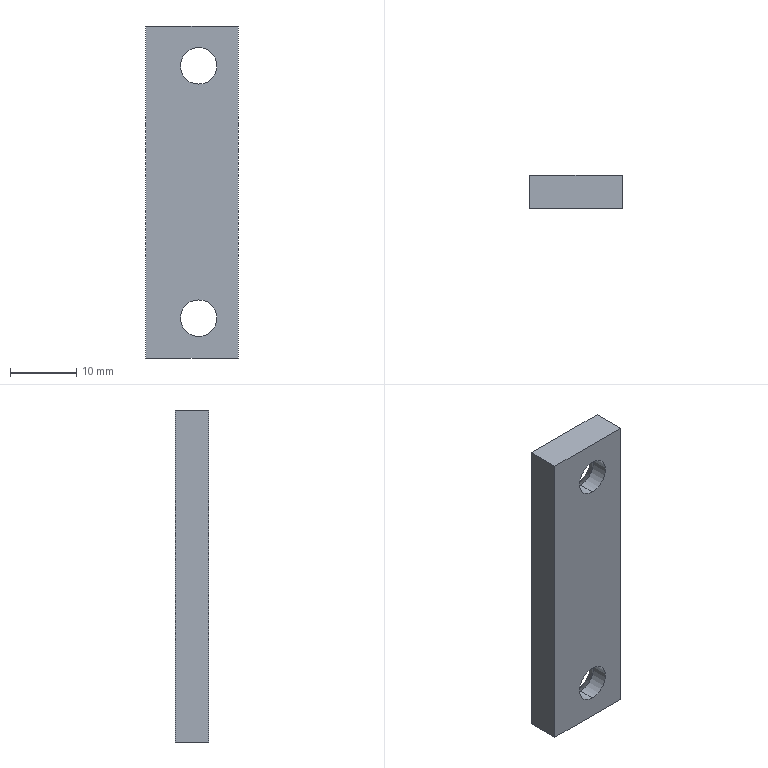Component | SolidWorks | PusherBlockSlideSeatCoverPlate3-1 | 1 solid | 14 faces | box 14 x 5 x 50 mm | volume 3128 mm3 | plane 6 | cone 4 | cylinder 4 | commonest cylinder face diameters 5.5 x4
build123d program:
from build123d import *

# Parameters (mm, degrees)
SKETCH1_W                                    = 50
SKETCH1_H                                    = 14
BOSS_EXTRUDE1_DEPTH                          = 5
TAPERED_COUNTERSUNK_HOLE_FOR_M5_FLAT_2_COUNT = 2
TAPERED_COUNTERSUNK_HOLE_FOR_M5_FLAT_2_PITCH = 38


with BuildPart() as part:
    # Sketch1 → Boss-Extrude1 (new body)
    with BuildSketch(Plane.XY):
        with Locations((-25, 7)):
            Rectangle(SKETCH1_W, SKETCH1_H)
    extrude(amount=BOSS_EXTRUDE1_DEPTH)

    # Sketch2 → Tapered Countersunk Hole for M5 Flat Hea (revolve, cut)
    with BuildSketch(Plane(origin=(-44, 6, 5), x_dir=(0, -1, 0), z_dir=(1, 0, 0))):
        Polygon((0, 0), (0, 5), (2.75, 5), (2.75, 2.45), (5.2, 0), align=None)
    tapered_countersunk_hole_for_m5_flat_hea = revolve(axis=Axis((-44, 6, 11.35), (0, 0, -1)), mode=Mode.SUBTRACT)

    # Tapered Countersunk Hole for M5 Flat 2: Tapered Countersunk Hole for M5 Flat Hea ×2
    with Locations(*[(i * TAPERED_COUNTERSUNK_HOLE_FOR_M5_FLAT_2_PITCH, 0, 0) for i in range(1, TAPERED_COUNTERSUNK_HOLE_FOR_M5_FLAT_2_COUNT)]):
        add(tapered_countersunk_hole_for_m5_flat_hea, mode=Mode.SUBTRACT)


solid = part.part

# Placed as in the assembly
solid = solid.moved(Location((22.085, 11.195, 51.579), (-90, 0, 90)))
STEP:
#1=COLOUR_RGB('',0.7922,0.8196,0.9333);
#2=FILL_AREA_STYLE_COLOUR('',#1);
#3=FILL_AREA_STYLE('',(#2));
#4=SURFACE_STYLE_FILL_AREA(#3);
#5=SURFACE_SIDE_STYLE('',(#4));
#6=SURFACE_STYLE_USAGE(.BOTH.,#5);
#7=PRESENTATION_STYLE_ASSIGNMENT((#6));
#8=CARTESIAN_POINT('',(0.6333,0.5411,3.871));
#9=VERTEX_POINT('',#8);
#10=CARTESIAN_POINT('',(0.6333,0.5411,3.655));
#11=VERTEX_POINT('',#10);
#12=CARTESIAN_POINT('',(0.6333,0.5411,3.763));
#13=DIRECTION('',(-0.,1.,-0.));
#14=DIRECTION('',(0.,0.,-1.));
#15=AXIS2_PLACEMENT_3D('',#12,#13,#14);
#16=CIRCLE('',#15,0.1083);
#17=EDGE_CURVE('',#9,#11,#16,.T.);
#18=ORIENTED_EDGE('',*,*,#17,.F.);
#19=CARTESIAN_POINT('',(0.6333,0.6376,3.968));
#20=VERTEX_POINT('',#19);
#21=CARTESIAN_POINT('',(0.6333,0.6376,3.968));
#22=DIRECTION('',(-0.,0.7071,0.7071));
#23=VECTOR('',#22,39.37);
#24=LINE('',#21,#23);
#25=EDGE_CURVE('',#9,#20,#24,.T.);
#26=ORIENTED_EDGE('',*,*,#25,.T.);
#27=CARTESIAN_POINT('',(0.6333,0.6376,3.558));
#28=VERTEX_POINT('',#27);
#29=CARTESIAN_POINT('',(0.6333,0.6376,3.763));
#30=DIRECTION('',(-0.,1.,-0.));
#31=DIRECTION('',(0.,0.,-1.));
#32=AXIS2_PLACEMENT_3D('',#29,#30,#31);
#33=CIRCLE('',#32,0.2047);
#34=EDGE_CURVE('',#20,#28,#33,.T.);
#35=ORIENTED_EDGE('',*,*,#34,.T.);
#36=CARTESIAN_POINT('',(0.6333,0.6376,3.558));
#37=DIRECTION('',(-0.,0.7071,-0.7071));
#38=VECTOR('',#37,39.37);
#39=LINE('',#36,#38);
#40=EDGE_CURVE('',#11,#28,#39,.T.);
#41=ORIENTED_EDGE('',*,*,#40,.F.);
#42=EDGE_LOOP('',(#18,#26,#35,#41));
#43=FACE_OUTER_BOUND('',#42,.T.);
#44=CARTESIAN_POINT('',(0.6333,0.6376,3.763));
#45=DIRECTION('',(-0.,1.,-0.));
#46=DIRECTION('',(0.,0.,-1.));
#47=AXIS2_PLACEMENT_3D('',#44,#45,#46);
#48=CONICAL_SURFACE('',#47,0.2047,0.7854);
#49=ADVANCED_FACE('',(#43),#48,.F.);
#50=CARTESIAN_POINT('',(0.6333,0.4407,3.871));
#51=VERTEX_POINT('',#50);
#52=CARTESIAN_POINT('',(0.6333,0.4407,3.655));
#53=VERTEX_POINT('',#52);
#54=CARTESIAN_POINT('',(0.6333,0.4407,3.763));
#55=DIRECTION('',(-0.,1.,-0.));
#56=DIRECTION('',(0.,0.,-1.));
#57=AXIS2_PLACEMENT_3D('',#54,#55,#56);
#58=CIRCLE('',#57,0.1083);
#59=EDGE_CURVE('',#51,#53,#58,.T.);
#60=ORIENTED_EDGE('',*,*,#59,.F.);
#61=CARTESIAN_POINT('',(0.6333,0.6376,3.871));
#62=DIRECTION('',(-0.,1.,-0.));
#63=VECTOR('',#62,39.37);
#64=LINE('',#61,#63);
#65=EDGE_CURVE('',#51,#9,#64,.T.);
#66=ORIENTED_EDGE('',*,*,#65,.T.);
#67=ORIENTED_EDGE('',*,*,#17,.T.);
#68=CARTESIAN_POINT('',(0.6333,0.6376,3.655));
#69=DIRECTION('',(-0.,1.,-0.));
#70=VECTOR('',#69,39.37);
#71=LINE('',#68,#70);
#72=EDGE_CURVE('',#53,#11,#71,.T.);
#73=ORIENTED_EDGE('',*,*,#72,.F.);
#74=EDGE_LOOP('',(#60,#66,#67,#73));
#75=FACE_OUTER_BOUND('',#74,.T.);
#76=CARTESIAN_POINT('',(0.6333,0.6376,3.763));
#77=DIRECTION('',(-0.,1.,-0.));
#78=DIRECTION('',(0.,0.,-1.));
#79=AXIS2_PLACEMENT_3D('',#76,#77,#78);
#80=CYLINDRICAL_SURFACE('',#79,0.1083);
#81=ADVANCED_FACE('',(#75),#80,.F.);
#82=CARTESIAN_POINT('',(0.6333,0.5411,2.375));
#83=VERTEX_POINT('',#82);
#84=CARTESIAN_POINT('',(0.6333,0.5411,2.159));
#85=VERTEX_POINT('',#84);
#86=CARTESIAN_POINT('',(0.6333,0.5411,2.267));
#87=DIRECTION('',(-0.,1.,-0.));
#88=DIRECTION('',(0.,0.,-1.));
#89=AXIS2_PLACEMENT_3D('',#86,#87,#88);
#90=CIRCLE('',#89,0.1083);
#91=EDGE_CURVE('',#83,#85,#90,.T.);
#92=ORIENTED_EDGE('',*,*,#91,.F.);
#93=CARTESIAN_POINT('',(0.6333,0.6376,2.472));
#94=VERTEX_POINT('',#93);
#95=CARTESIAN_POINT('',(0.6333,0.6376,2.472));
#96=DIRECTION('',(-0.,0.7071,0.7071));
#97=VECTOR('',#96,39.37);
#98=LINE('',#95,#97);
#99=EDGE_CURVE('',#83,#94,#98,.T.);
#100=ORIENTED_EDGE('',*,*,#99,.T.);
#101=CARTESIAN_POINT('',(0.6333,0.6376,2.062));
#102=VERTEX_POINT('',#101);
#103=CARTESIAN_POINT('',(0.6333,0.6376,2.267));
#104=DIRECTION('',(-0.,1.,-0.));
#105=DIRECTION('',(0.,0.,-1.));
#106=AXIS2_PLACEMENT_3D('',#103,#104,#105);
#107=CIRCLE('',#106,0.2047);
#108=EDGE_CURVE('',#94,#102,#107,.T.);
#109=ORIENTED_EDGE('',*,*,#108,.T.);
#110=CARTESIAN_POINT('',(0.6333,0.6376,2.062));
#111=DIRECTION('',(-0.,0.7071,-0.7071));
#112=VECTOR('',#111,39.37);
#113=LINE('',#110,#112);
#114=EDGE_CURVE('',#85,#102,#113,.T.);
#115=ORIENTED_EDGE('',*,*,#114,.F.);
#116=EDGE_LOOP('',(#92,#100,#109,#115));
#117=FACE_OUTER_BOUND('',#116,.T.);
#118=CARTESIAN_POINT('',(0.6333,0.6376,2.267));
#119=DIRECTION('',(-0.,1.,-0.));
#120=DIRECTION('',(0.,0.,-1.));
#121=AXIS2_PLACEMENT_3D('',#118,#119,#120);
#122=CONICAL_SURFACE('',#121,0.2047,0.7854);
#123=ADVANCED_FACE('',(#117),#122,.F.);
#124=CARTESIAN_POINT('',(0.6333,0.4407,2.375));
#125=VERTEX_POINT('',#124);
#126=CARTESIAN_POINT('',(0.6333,0.4407,2.159));
#127=VERTEX_POINT('',#126);
#128=CARTESIAN_POINT('',(0.6333,0.4407,2.267));
#129=DIRECTION('',(-0.,1.,-0.));
#130=DIRECTION('',(0.,0.,-1.));
#131=AXIS2_PLACEMENT_3D('',#128,#129,#130);
#132=CIRCLE('',#131,0.1083);
#133=EDGE_CURVE('',#125,#127,#132,.T.);
#134=ORIENTED_EDGE('',*,*,#133,.F.);
#135=CARTESIAN_POINT('',(0.6333,0.6376,2.375));
#136=DIRECTION('',(-0.,1.,-0.));
#137=VECTOR('',#136,39.37);
#138=LINE('',#135,#137);
#139=EDGE_CURVE('',#125,#83,#138,.T.);
#140=ORIENTED_EDGE('',*,*,#139,.T.);
#141=ORIENTED_EDGE('',*,*,#91,.T.);
#142=CARTESIAN_POINT('',(0.6333,0.6376,2.159));
#143=DIRECTION('',(-0.,1.,-0.));
#144=VECTOR('',#143,39.37);
#145=LINE('',#142,#144);
#146=EDGE_CURVE('',#127,#85,#145,.T.);
#147=ORIENTED_EDGE('',*,*,#146,.F.);
#148=EDGE_LOOP('',(#134,#140,#141,#147));
#149=FACE_OUTER_BOUND('',#148,.T.);
#150=CARTESIAN_POINT('',(0.6333,0.6376,2.267));
#151=DIRECTION('',(-0.,1.,-0.));
#152=DIRECTION('',(0.,0.,-1.));
#153=AXIS2_PLACEMENT_3D('',#150,#151,#152);
#154=CYLINDRICAL_SURFACE('',#153,0.1083);
#155=ADVANCED_FACE('',(#149),#154,.F.);
#156=CARTESIAN_POINT('',(0.8695,0.4407,2.031));
#157=VERTEX_POINT('',#156);
#158=CARTESIAN_POINT('',(0.3183,0.4407,2.031));
#159=VERTEX_POINT('',#158);
#160=CARTESIAN_POINT('',(0.8695,0.4407,2.031));
#161=DIRECTION('',(-1.,0.,0.));
#162=VECTOR('',#161,39.37);
#163=LINE('',#160,#162);
#164=EDGE_CURVE('',#157,#159,#163,.T.);
#165=ORIENTED_EDGE('',*,*,#164,.T.);
#166=CARTESIAN_POINT('',(0.3183,0.6376,2.031));
#167=VERTEX_POINT('',#166);
#168=CARTESIAN_POINT('',(0.3183,0.6376,2.031));
#169=DIRECTION('',(0.,-1.,0.));
#170=VECTOR('',#169,39.37);
#171=LINE('',#168,#170);
#172=EDGE_CURVE('',#167,#159,#171,.T.);
#173=ORIENTED_EDGE('',*,*,#172,.F.);
#174=CARTESIAN_POINT('',(0.8695,0.6376,2.031));
#175=VERTEX_POINT('',#174);
#176=CARTESIAN_POINT('',(0.8695,0.6376,2.031));
#177=DIRECTION('',(-1.,0.,0.));
#178=VECTOR('',#177,39.37);
#179=LINE('',#176,#178);
#180=EDGE_CURVE('',#175,#167,#179,.T.);
#181=ORIENTED_EDGE('',*,*,#180,.F.);
#182=CARTESIAN_POINT('',(0.8695,0.6376,2.031));
#183=DIRECTION('',(0.,-1.,0.));
#184=VECTOR('',#183,39.37);
#185=LINE('',#182,#184);
#186=EDGE_CURVE('',#175,#157,#185,.T.);
#187=ORIENTED_EDGE('',*,*,#186,.T.);
#188=EDGE_LOOP('',(#165,#173,#181,#187));
#189=FACE_OUTER_BOUND('',#188,.T.);
#190=CARTESIAN_POINT('',(0.8695,0.6376,2.031));
#191=DIRECTION('',(0.,0.,1.));
#192=DIRECTION('',(-0.,1.,-0.));
#193=AXIS2_PLACEMENT_3D('',#190,#191,#192);
#194=PLANE('',#193);
#195=ADVANCED_FACE('',(#189),#194,.F.);
#196=CARTESIAN_POINT('',(0.3183,0.4407,3.999));
#197=VERTEX_POINT('',#196);
#198=CARTESIAN_POINT('',(0.3183,0.4407,2.031));
#199=DIRECTION('',(0.,-0.,1.));
#200=VECTOR('',#199,39.37);
#201=LINE('',#198,#200);
#202=EDGE_CURVE('',#159,#197,#201,.T.);
#203=ORIENTED_EDGE('',*,*,#202,.T.);
#204=CARTESIAN_POINT('',(0.3183,0.6376,3.999));
#205=VERTEX_POINT('',#204);
#206=CARTESIAN_POINT('',(0.3183,0.6376,3.999));
#207=DIRECTION('',(0.,-1.,0.));
#208=VECTOR('',#207,39.37);
#209=LINE('',#206,#208);
#210=EDGE_CURVE('',#205,#197,#209,.T.);
#211=ORIENTED_EDGE('',*,*,#210,.F.);
#212=CARTESIAN_POINT('',(0.3183,0.6376,2.031));
#213=DIRECTION('',(0.,-0.,1.));
#214=VECTOR('',#213,39.37);
#215=LINE('',#212,#214);
#216=EDGE_CURVE('',#167,#205,#215,.T.);
#217=ORIENTED_EDGE('',*,*,#216,.F.);
#218=ORIENTED_EDGE('',*,*,#172,.T.);
#219=EDGE_LOOP('',(#203,#211,#217,#218));
#220=FACE_OUTER_BOUND('',#219,.T.);
#221=CARTESIAN_POINT('',(0.3183,0.6376,2.031));
#222=DIRECTION('',(1.,-0.,-0.));
#223=DIRECTION('',(-0.,0.,-1.));
#224=AXIS2_PLACEMENT_3D('',#221,#222,#223);
#225=PLANE('',#224);
#226=ADVANCED_FACE('',(#220),#225,.F.);
#227=CARTESIAN_POINT('',(0.8695,0.4407,3.999));
#228=VERTEX_POINT('',#227);
#229=CARTESIAN_POINT('',(0.8695,0.4407,3.999));
#230=DIRECTION('',(1.,-0.,-0.));
#231=VECTOR('',#230,39.37);
#232=LINE('',#229,#231);
#233=EDGE_CURVE('',#197,#228,#232,.T.);
#234=ORIENTED_EDGE('',*,*,#233,.T.);
#235=CARTESIAN_POINT('',(0.8695,0.6376,3.999));
#236=VERTEX_POINT('',#235);
#237=CARTESIAN_POINT('',(0.8695,0.6376,3.999));
#238=DIRECTION('',(0.,-1.,0.));
#239=VECTOR('',#238,39.37);
#240=LINE('',#237,#239);
#241=EDGE_CURVE('',#236,#228,#240,.T.);
#242=ORIENTED_EDGE('',*,*,#241,.F.);
#243=CARTESIAN_POINT('',(0.8695,0.6376,3.999));
#244=DIRECTION('',(1.,-0.,-0.));
#245=VECTOR('',#244,39.37);
#246=LINE('',#243,#245);
#247=EDGE_CURVE('',#205,#236,#246,.T.);
#248=ORIENTED_EDGE('',*,*,#247,.F.);
#249=ORIENTED_EDGE('',*,*,#210,.T.);
#250=EDGE_LOOP('',(#234,#242,#248,#249));
#251=FACE_OUTER_BOUND('',#250,.T.);
#252=CARTESIAN_POINT('',(0.8695,0.6376,3.999));
#253=DIRECTION('',(-0.,-0.,-1.));
#254=DIRECTION('',(0.,-1.,0.));
#255=AXIS2_PLACEMENT_3D('',#252,#253,#254);
#256=PLANE('',#255);
#257=ADVANCED_FACE('',(#251),#256,.F.);
#258=CARTESIAN_POINT('',(0.8695,0.4407,2.031));
#259=DIRECTION('',(-0.,0.,-1.));
#260=VECTOR('',#259,39.37);
#261=LINE('',#258,#260);
#262=EDGE_CURVE('',#228,#157,#261,.T.);
#263=ORIENTED_EDGE('',*,*,#262,.T.);
#264=ORIENTED_EDGE('',*,*,#186,.F.);
#265=CARTESIAN_POINT('',(0.8695,0.6376,2.031));
#266=DIRECTION('',(-0.,0.,-1.));
#267=VECTOR('',#266,39.37);
#268=LINE('',#265,#267);
#269=EDGE_CURVE('',#236,#175,#268,.T.);
#270=ORIENTED_EDGE('',*,*,#269,.F.);
#271=ORIENTED_EDGE('',*,*,#241,.T.);
#272=EDGE_LOOP('',(#263,#264,#270,#271));
#273=FACE_OUTER_BOUND('',#272,.T.);
#274=CARTESIAN_POINT('',(0.8695,0.6376,2.031));
#275=DIRECTION('',(-1.,0.,0.));
#276=DIRECTION('',(0.,-0.,1.));
#277=AXIS2_PLACEMENT_3D('',#274,#275,#276);
#278=PLANE('',#277);
#279=ADVANCED_FACE('',(#273),#278,.F.);
#280=CARTESIAN_POINT('',(0.6333,0.6376,3.763));
#281=DIRECTION('',(-0.,1.,-0.));
#282=DIRECTION('',(0.,0.,-1.));
#283=AXIS2_PLACEMENT_3D('',#280,#281,#282);
#284=CIRCLE('',#283,0.2047);
#285=EDGE_CURVE('',#28,#20,#284,.T.);
#286=ORIENTED_EDGE('',*,*,#285,.F.);
#287=ORIENTED_EDGE('',*,*,#34,.F.);
#288=EDGE_LOOP('',(#286,#287));
#289=FACE_BOUND('',#288,.T.);
#290=CARTESIAN_POINT('',(0.6333,0.6376,2.267));
#291=DIRECTION('',(-0.,1.,-0.));
#292=DIRECTION('',(0.,0.,-1.));
#293=AXIS2_PLACEMENT_3D('',#290,#291,#292);
#294=CIRCLE('',#293,0.2047);
#295=EDGE_CURVE('',#102,#94,#294,.T.);
#296=ORIENTED_EDGE('',*,*,#295,.F.);
#297=ORIENTED_EDGE('',*,*,#108,.F.);
#298=EDGE_LOOP('',(#296,#297));
#299=FACE_BOUND('',#298,.T.);
#300=ORIENTED_EDGE('',*,*,#180,.T.);
#301=ORIENTED_EDGE('',*,*,#216,.T.);
#302=ORIENTED_EDGE('',*,*,#247,.T.);
#303=ORIENTED_EDGE('',*,*,#269,.T.);
#304=EDGE_LOOP('',(#300,#301,#302,#303));
#305=FACE_OUTER_BOUND('',#304,.T.);
#306=CARTESIAN_POINT('',(0.3183,0.6376,2.031));
#307=DIRECTION('',(-0.,1.,0.));
#308=DIRECTION('',(-0.,0.,-1.));
#309=AXIS2_PLACEMENT_3D('',#306,#307,#308);
#310=PLANE('',#309);
#311=ADVANCED_FACE('',(#289,#299,#305),#310,.T.);
#312=CARTESIAN_POINT('',(0.6333,0.4407,3.763));
#313=DIRECTION('',(-0.,1.,-0.));
#314=DIRECTION('',(0.,0.,-1.));
#315=AXIS2_PLACEMENT_3D('',#312,#313,#314);
#316=CIRCLE('',#315,0.1083);
#317=EDGE_CURVE('',#53,#51,#316,.T.);
#318=ORIENTED_EDGE('',*,*,#317,.T.);
#319=ORIENTED_EDGE('',*,*,#59,.T.);
#320=EDGE_LOOP('',(#318,#319));
#321=FACE_BOUND('',#320,.T.);
#322=CARTESIAN_POINT('',(0.6333,0.4407,2.267));
#323=DIRECTION('',(-0.,1.,-0.));
#324=DIRECTION('',(0.,0.,-1.));
#325=AXIS2_PLACEMENT_3D('',#322,#323,#324);
#326=CIRCLE('',#325,0.1083);
#327=EDGE_CURVE('',#127,#125,#326,.T.);
#328=ORIENTED_EDGE('',*,*,#327,.T.);
#329=ORIENTED_EDGE('',*,*,#133,.T.);
#330=EDGE_LOOP('',(#328,#329));
#331=FACE_BOUND('',#330,.T.);
#332=ORIENTED_EDGE('',*,*,#164,.F.);
#333=ORIENTED_EDGE('',*,*,#262,.F.);
#334=ORIENTED_EDGE('',*,*,#233,.F.);
#335=ORIENTED_EDGE('',*,*,#202,.F.);
#336=EDGE_LOOP('',(#332,#333,#334,#335));
#337=FACE_OUTER_BOUND('',#336,.T.);
#338=CARTESIAN_POINT('',(0.3183,0.4407,2.031));
#339=DIRECTION('',(-0.,1.,0.));
#340=DIRECTION('',(-0.,0.,-1.));
#341=AXIS2_PLACEMENT_3D('',#338,#339,#340);
#342=PLANE('',#341);
#343=ADVANCED_FACE('',(#321,#331,#337),#342,.F.);
#344=ORIENTED_EDGE('',*,*,#139,.F.);
#345=ORIENTED_EDGE('',*,*,#327,.F.);
#346=ORIENTED_EDGE('',*,*,#146,.T.);
#347=CARTESIAN_POINT('',(0.6333,0.5411,2.267));
#348=DIRECTION('',(-0.,1.,-0.));
#349=DIRECTION('',(0.,0.,-1.));
#350=AXIS2_PLACEMENT_3D('',#347,#348,#349);
#351=CIRCLE('',#350,0.1083);
#352=EDGE_CURVE('',#85,#83,#351,.T.);
#353=ORIENTED_EDGE('',*,*,#352,.T.);
#354=EDGE_LOOP('',(#344,#345,#346,#353));
#355=FACE_OUTER_BOUND('',#354,.T.);
#356=CARTESIAN_POINT('',(0.6333,0.6376,2.267));
#357=DIRECTION('',(-0.,1.,-0.));
#358=DIRECTION('',(0.,0.,-1.));
#359=AXIS2_PLACEMENT_3D('',#356,#357,#358);
#360=CYLINDRICAL_SURFACE('',#359,0.1083);
#361=ADVANCED_FACE('',(#355),#360,.F.);
#362=ORIENTED_EDGE('',*,*,#99,.F.);
#363=ORIENTED_EDGE('',*,*,#352,.F.);
#364=ORIENTED_EDGE('',*,*,#114,.T.);
#365=ORIENTED_EDGE('',*,*,#295,.T.);
#366=EDGE_LOOP('',(#362,#363,#364,#365));
#367=FACE_OUTER_BOUND('',#366,.T.);
#368=CARTESIAN_POINT('',(0.6333,0.6376,2.267));
#369=DIRECTION('',(-0.,1.,-0.));
#370=DIRECTION('',(0.,0.,-1.));
#371=AXIS2_PLACEMENT_3D('',#368,#369,#370);
#372=CONICAL_SURFACE('',#371,0.2047,0.7854);
#373=ADVANCED_FACE('',(#367),#372,.F.);
#374=ORIENTED_EDGE('',*,*,#65,.F.);
#375=ORIENTED_EDGE('',*,*,#317,.F.);
#376=ORIENTED_EDGE('',*,*,#72,.T.);
#377=CARTESIAN_POINT('',(0.6333,0.5411,3.763));
#378=DIRECTION('',(-0.,1.,-0.));
#379=DIRECTION('',(0.,0.,-1.));
#380=AXIS2_PLACEMENT_3D('',#377,#378,#379);
#381=CIRCLE('',#380,0.1083);
#382=EDGE_CURVE('',#11,#9,#381,.T.);
#383=ORIENTED_EDGE('',*,*,#382,.T.);
#384=EDGE_LOOP('',(#374,#375,#376,#383));
#385=FACE_OUTER_BOUND('',#384,.T.);
#386=CARTESIAN_POINT('',(0.6333,0.6376,3.763));
#387=DIRECTION('',(-0.,1.,-0.));
#388=DIRECTION('',(0.,0.,-1.));
#389=AXIS2_PLACEMENT_3D('',#386,#387,#388);
#390=CYLINDRICAL_SURFACE('',#389,0.1083);
#391=ADVANCED_FACE('',(#385),#390,.F.);
#392=ORIENTED_EDGE('',*,*,#25,.F.);
#393=ORIENTED_EDGE('',*,*,#382,.F.);
#394=ORIENTED_EDGE('',*,*,#40,.T.);
#395=ORIENTED_EDGE('',*,*,#285,.T.);
#396=EDGE_LOOP('',(#392,#393,#394,#395));
#397=FACE_OUTER_BOUND('',#396,.T.);
#398=CARTESIAN_POINT('',(0.6333,0.6376,3.763));
#399=DIRECTION('',(-0.,1.,-0.));
#400=DIRECTION('',(0.,0.,-1.));
#401=AXIS2_PLACEMENT_3D('',#398,#399,#400);
#402=CONICAL_SURFACE('',#401,0.2047,0.7854);
#403=ADVANCED_FACE('',(#397),#402,.F.);
#404=CLOSED_SHELL('',(#49,#81,#123,#155,#195,#226,#257,#279,#311,#343,#361,#373,#391,#403));
#405=MANIFOLD_SOLID_BREP('',#404);
#406=STYLED_ITEM('',(#7),#405);
#407=PRESENTATION_LAYER_ASSIGNMENT('','',(#406));
#408=(LENGTH_UNIT()NAMED_UNIT(*)SI_UNIT($,.METRE.));
#409=LENGTH_MEASURE_WITH_UNIT(LENGTH_MEASURE(0.0254),#408);
#410=DIMENSIONAL_EXPONENTS(1.,0.,0.,0.,0.,0.,0.);
#411=(CONVERSION_BASED_UNIT('',#409)LENGTH_UNIT()NAMED_UNIT(#410));
#412=UNCERTAINTY_MEASURE_WITH_UNIT(LENGTH_MEASURE(0.00001),#411,'','');
#413=(NAMED_UNIT(*)PLANE_ANGLE_UNIT()SI_UNIT($,.RADIAN.));
#414=(NAMED_UNIT(*)SI_UNIT($,.STERADIAN.)SOLID_ANGLE_UNIT());
#415=(GEOMETRIC_REPRESENTATION_CONTEXT(3)GLOBAL_UNCERTAINTY_ASSIGNED_CONTEXT((#412))GLOBAL_UNIT_ASSIGNED_CONTEXT((#411,#413,#414))REPRESENTATION_CONTEXT('',''));
#416=MECHANICAL_DESIGN_GEOMETRIC_PRESENTATION_REPRESENTATION('',(#406),#415);
#417=CARTESIAN_POINT('',(0.,0.,0.));
#418=DIRECTION('',(0.,0.,1.));
#419=DIRECTION('',(1.,0.,0.));
#420=AXIS2_PLACEMENT_3D('',#417,#418,#419);
#421=(LENGTH_UNIT()NAMED_UNIT(*)SI_UNIT($,.METRE.));
#422=LENGTH_MEASURE_WITH_UNIT(LENGTH_MEASURE(0.0254),#421);
#423=DIMENSIONAL_EXPONENTS(1.,0.,0.,0.,0.,0.,0.);
#424=(CONVERSION_BASED_UNIT('',#422)LENGTH_UNIT()NAMED_UNIT(#423));
#425=UNCERTAINTY_MEASURE_WITH_UNIT(LENGTH_MEASURE(0.00001),#424,'','');
#426=(NAMED_UNIT(*)PLANE_ANGLE_UNIT()SI_UNIT($,.RADIAN.));
#427=(NAMED_UNIT(*)SI_UNIT($,.STERADIAN.)SOLID_ANGLE_UNIT());
#428=(GEOMETRIC_REPRESENTATION_CONTEXT(3)GLOBAL_UNCERTAINTY_ASSIGNED_CONTEXT((#425))GLOBAL_UNIT_ASSIGNED_CONTEXT((#424,#426,#427))REPRESENTATION_CONTEXT('',''));
#429=ADVANCED_BREP_SHAPE_REPRESENTATION('',(#405,#420),#428);